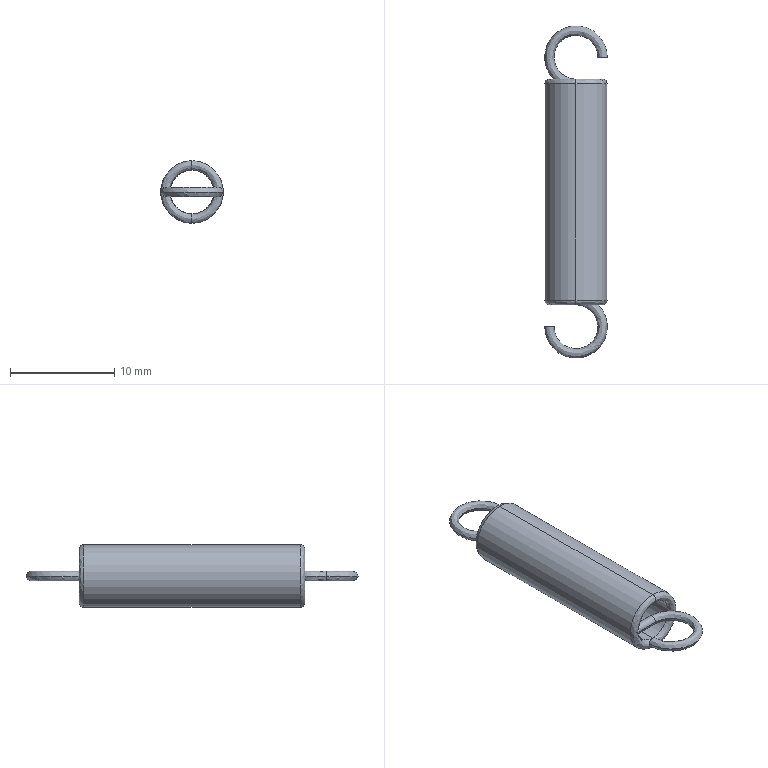Component | SolidWorks | YAWF-D6-L30-1 | 1 solid | 18 faces | box 6 x 31.8 x 6 mm | volume 327 mm3 | spline 8 | cylinder 8 | plane 2 | commonest cylinder face diameters 0.9 x4 6 x2 4.2 x2 | material Purchased Part
STEP:
#1=CARTESIAN_POINT('',(-2.205,-1.423,-0.001969));
#2=VERTEX_POINT('',#1);
#3=CARTESIAN_POINT('',(-2.124,-1.423,0.06299));
#4=VERTEX_POINT('',#3);
#5=CARTESIAN_POINT('',(-2.124,-1.423,-0.01969));
#6=DIRECTION('',(-0.,1.,-0.));
#7=DIRECTION('',(0.,0.,-1.));
#8=AXIS2_PLACEMENT_3D('',#5,#6,#7);
#9=CIRCLE('',#8,0.08268);
#10=EDGE_CURVE('',#2,#4,#9,.T.);
#11=ORIENTED_EDGE('',*,*,#10,.T.);
#12=CARTESIAN_POINT('',(-2.124,-1.423,0.09843));
#13=VERTEX_POINT('',#12);
#14=CARTESIAN_POINT('',(-2.124,-1.423,0.08071));
#15=DIRECTION('',(-1.,-0.,0.));
#16=DIRECTION('',(0.,0.,1.));
#17=AXIS2_PLACEMENT_3D('',#14,#15,#16);
#18=CIRCLE('',#17,0.01772);
#19=EDGE_CURVE('',#4,#13,#18,.T.);
#20=ORIENTED_EDGE('',*,*,#19,.T.);
#21=CARTESIAN_POINT('',(-2.124,-1.423,-0.1378));
#22=VERTEX_POINT('',#21);
#23=CARTESIAN_POINT('',(-2.124,-1.423,-0.01969));
#24=DIRECTION('',(-0.,1.,-0.));
#25=DIRECTION('',(0.,0.,1.));
#26=AXIS2_PLACEMENT_3D('',#23,#24,#25);
#27=CIRCLE('',#26,0.1181);
#28=EDGE_CURVE('',#22,#13,#27,.T.);
#29=ORIENTED_EDGE('',*,*,#28,.F.);
#30=CARTESIAN_POINT('',(-2.124,-1.423,-0.1024));
#31=VERTEX_POINT('',#30);
#32=CARTESIAN_POINT('',(-2.124,-1.423,-0.1201));
#33=DIRECTION('',(1.,-0.,0.));
#34=DIRECTION('',(0.,0.,-1.));
#35=AXIS2_PLACEMENT_3D('',#32,#33,#34);
#36=CIRCLE('',#35,0.01772);
#37=EDGE_CURVE('',#31,#22,#36,.T.);
#38=ORIENTED_EDGE('',*,*,#37,.F.);
#39=CARTESIAN_POINT('',(-2.205,-1.423,-0.0374));
#40=VERTEX_POINT('',#39);
#41=CARTESIAN_POINT('',(-2.124,-1.423,-0.01969));
#42=DIRECTION('',(-0.,1.,-0.));
#43=DIRECTION('',(0.,0.,-1.));
#44=AXIS2_PLACEMENT_3D('',#41,#42,#43);
#45=CIRCLE('',#44,0.08268);
#46=EDGE_CURVE('',#31,#40,#45,.T.);
#47=ORIENTED_EDGE('',*,*,#46,.T.);
#48=CARTESIAN_POINT('',(-2.224,-1.441,-0.01969));
#49=VERTEX_POINT('',#48);
#50=CARTESIAN_POINT('',(-2.205,-1.423,-0.0374));
#51=CARTESIAN_POINT('',(-2.205,-1.425,-0.0374));
#52=CARTESIAN_POINT('',(-2.205,-1.426,-0.03725));
#53=CARTESIAN_POINT('',(-2.206,-1.428,-0.03677));
#54=CARTESIAN_POINT('',(-2.206,-1.429,-0.03657));
#55=CARTESIAN_POINT('',(-2.206,-1.43,-0.03621));
#56=CARTESIAN_POINT('',(-2.206,-1.43,-0.03602));
#57=CARTESIAN_POINT('',(-2.207,-1.431,-0.03579));
#58=CARTESIAN_POINT('',(-2.207,-1.431,-0.03564));
#59=CARTESIAN_POINT('',(-2.207,-1.431,-0.03554));
#60=CARTESIAN_POINT('',(-2.208,-1.432,-0.03501));
#61=CARTESIAN_POINT('',(-2.208,-1.433,-0.03443));
#62=CARTESIAN_POINT('',(-2.21,-1.435,-0.03335));
#63=CARTESIAN_POINT('',(-2.21,-1.435,-0.03296));
#64=CARTESIAN_POINT('',(-2.211,-1.436,-0.03231));
#65=CARTESIAN_POINT('',(-2.211,-1.436,-0.03198));
#66=CARTESIAN_POINT('',(-2.212,-1.436,-0.03156));
#67=CARTESIAN_POINT('',(-2.212,-1.437,-0.03137));
#68=CARTESIAN_POINT('',(-2.212,-1.437,-0.03125));
#69=CARTESIAN_POINT('',(-2.212,-1.437,-0.03116));
#70=CARTESIAN_POINT('',(-2.213,-1.437,-0.03059));
#71=CARTESIAN_POINT('',(-2.214,-1.438,-0.02989));
#72=CARTESIAN_POINT('',(-2.215,-1.439,-0.02855));
#73=CARTESIAN_POINT('',(-2.216,-1.439,-0.02805));
#74=CARTESIAN_POINT('',(-2.217,-1.439,-0.02695));
#75=CARTESIAN_POINT('',(-2.218,-1.44,-0.0263));
#76=CARTESIAN_POINT('',(-2.221,-1.441,-0.02323));
#77=CARTESIAN_POINT('',(-2.223,-1.441,-0.02116));
#78=CARTESIAN_POINT('',(-2.224,-1.441,-0.01969));
#79=B_SPLINE_CURVE_WITH_KNOTS('',3,(#50,#51,#52,#53,#54,#55,#56,#57,#58,#59,#60,#61,#62,#63,#64,#65,#66,#67,#68,#69,#70,#71,#72,#73,#74,#75,#76,#77,#78),.UNSPECIFIED.,.F.,.F.,(4,2,2,1,2,2,2,2,1,1,2,2,2,2,2,4),(0.,0.125,0.1875,0.2187,0.2344,0.25,0.375,0.4375,0.4687,0.4844,0.4922,0.5,0.625,0.6875,0.75,1.),.UNSPECIFIED.);
#80=EDGE_CURVE('',#40,#49,#79,.T.);
#81=ORIENTED_EDGE('',*,*,#80,.T.);
#82=CARTESIAN_POINT('',(-2.224,-1.441,-0.01969));
#83=CARTESIAN_POINT('',(-2.224,-1.441,-0.01895));
#84=CARTESIAN_POINT('',(-2.223,-1.441,-0.01806));
#85=CARTESIAN_POINT('',(-2.221,-1.441,-0.01655));
#86=CARTESIAN_POINT('',(-2.221,-1.441,-0.01602));
#87=CARTESIAN_POINT('',(-2.219,-1.44,-0.01489));
#88=CARTESIAN_POINT('',(-2.219,-1.44,-0.01436));
#89=CARTESIAN_POINT('',(-2.217,-1.439,-0.01236));
#90=CARTESIAN_POINT('',(-2.216,-1.439,-0.01127));
#91=CARTESIAN_POINT('',(-2.214,-1.438,-0.009926));
#92=CARTESIAN_POINT('',(-2.214,-1.438,-0.009528));
#93=CARTESIAN_POINT('',(-2.213,-1.437,-0.009001));
#94=CARTESIAN_POINT('',(-2.213,-1.437,-0.008755));
#95=CARTESIAN_POINT('',(-2.213,-1.437,-0.008497));
#96=CARTESIAN_POINT('',(-2.212,-1.437,-0.008393));
#97=CARTESIAN_POINT('',(-2.212,-1.437,-0.008325));
#98=CARTESIAN_POINT('',(-2.212,-1.437,-0.008322));
#99=CARTESIAN_POINT('',(-2.211,-1.436,-0.007245));
#100=CARTESIAN_POINT('',(-2.21,-1.435,-0.006391));
#101=CARTESIAN_POINT('',(-2.209,-1.434,-0.005311));
#102=CARTESIAN_POINT('',(-2.208,-1.433,-0.004985));
#103=CARTESIAN_POINT('',(-2.208,-1.432,-0.004543));
#104=CARTESIAN_POINT('',(-2.208,-1.432,-0.004334));
#105=CARTESIAN_POINT('',(-2.207,-1.432,-0.004142));
#106=CARTESIAN_POINT('',(-2.207,-1.432,-0.004018));
#107=CARTESIAN_POINT('',(-2.207,-1.431,-0.003982));
#108=CARTESIAN_POINT('',(-2.206,-1.429,-0.002578));
#109=CARTESIAN_POINT('',(-2.205,-1.426,-0.001969));
#110=CARTESIAN_POINT('',(-2.205,-1.423,-0.001969));
#111=B_SPLINE_CURVE_WITH_KNOTS('',3,(#82,#83,#84,#85,#86,#87,#88,#89,#90,#91,#92,#93,#94,#95,#96,#97,#98,#99,#100,#101,#102,#103,#104,#105,#106,#107,#108,#109,#110),.UNSPECIFIED.,.F.,.F.,(4,2,2,2,2,2,1,1,2,2,2,2,1,2,2,4),(0.,0.125,0.1875,0.25,0.375,0.4375,0.4688,0.4844,0.4922,0.5,0.625,0.6875,0.7188,0.7344,0.75,1.),.UNSPECIFIED.);
#112=EDGE_CURVE('',#49,#2,#111,.T.);
#113=ORIENTED_EDGE('',*,*,#112,.T.);
#114=EDGE_LOOP('',(#11,#20,#29,#38,#47,#81,#113));
#115=FACE_OUTER_BOUND('',#114,.T.);
#116=CARTESIAN_POINT('',(-2.124,-1.423,0.06299));
#117=CARTESIAN_POINT('',(-2.289,-1.423,0.06299));
#118=CARTESIAN_POINT('',(-2.289,-1.423,-0.1024));
#119=CARTESIAN_POINT('',(-2.124,-1.423,-0.1024));
#120=CARTESIAN_POINT('',(-2.124,-1.434,0.06299));
#121=CARTESIAN_POINT('',(-2.289,-1.434,0.06299));
#122=CARTESIAN_POINT('',(-2.289,-1.434,-0.1024));
#123=CARTESIAN_POINT('',(-2.124,-1.434,-0.1024));
#124=CARTESIAN_POINT('',(-2.124,-1.441,0.07033));
#125=CARTESIAN_POINT('',(-2.304,-1.441,0.07033));
#126=CARTESIAN_POINT('',(-2.304,-1.441,-0.1097));
#127=CARTESIAN_POINT('',(-2.124,-1.441,-0.1097));
#128=CARTESIAN_POINT('',(-2.124,-1.441,0.08071));
#129=CARTESIAN_POINT('',(-2.325,-1.441,0.08071));
#130=CARTESIAN_POINT('',(-2.325,-1.441,-0.1201));
#131=CARTESIAN_POINT('',(-2.124,-1.441,-0.1201));
#132=CARTESIAN_POINT('',(-2.124,-1.441,0.09109));
#133=CARTESIAN_POINT('',(-2.346,-1.441,0.09109));
#134=CARTESIAN_POINT('',(-2.346,-1.441,-0.1305));
#135=CARTESIAN_POINT('',(-2.124,-1.441,-0.1305));
#136=CARTESIAN_POINT('',(-2.124,-1.434,0.09843));
#137=CARTESIAN_POINT('',(-2.36,-1.434,0.09843));
#138=CARTESIAN_POINT('',(-2.36,-1.434,-0.1378));
#139=CARTESIAN_POINT('',(-2.124,-1.434,-0.1378));
#140=CARTESIAN_POINT('',(-2.124,-1.423,0.09843));
#141=CARTESIAN_POINT('',(-2.36,-1.423,0.09843));
#142=CARTESIAN_POINT('',(-2.36,-1.423,-0.1378));
#143=CARTESIAN_POINT('',(-2.124,-1.423,-0.1378));
#144=(BOUNDED_SURFACE()B_SPLINE_SURFACE(3,3,((#116,#117,#118,#119),(#120,#121,#122,#123),(#124,#125,#126,#127),(#128,#129,#130,#131),(#132,#133,#134,#135),(#136,#137,#138,#139),(#140,#141,#142,#143)),.UNSPECIFIED.,.F.,.F.,.F.)B_SPLINE_SURFACE_WITH_KNOTS((4,3,4),(4,4),(0.,0.5,1.),(0.,1.),.UNSPECIFIED.)GEOMETRIC_REPRESENTATION_ITEM()RATIONAL_B_SPLINE_SURFACE(((1.,0.3333,0.3333,1.),(0.8047,0.2682,0.2682,0.8047),(0.8047,0.2682,0.2682,0.8047),(1.,0.3333,0.3333,1.),(0.8047,0.2682,0.2682,0.8047),(0.8047,0.2682,0.2682,0.8047),(1.,0.3333,0.3333,1.)))REPRESENTATION_ITEM('')SURFACE());
#145=ADVANCED_FACE('',(#115),#144,.T.);
#146=CARTESIAN_POINT('',(-2.124,-0.6083,0.09843));
#147=VERTEX_POINT('',#146);
#148=CARTESIAN_POINT('',(-2.124,-0.6083,-0.1378));
#149=VERTEX_POINT('',#148);
#150=CARTESIAN_POINT('',(-2.124,-0.6083,-0.01969));
#151=DIRECTION('',(0.,-1.,0.));
#152=DIRECTION('',(0.,0.,1.));
#153=AXIS2_PLACEMENT_3D('',#150,#151,#152);
#154=CIRCLE('',#153,0.1181);
#155=EDGE_CURVE('',#147,#149,#154,.T.);
#156=ORIENTED_EDGE('',*,*,#155,.F.);
#157=CARTESIAN_POINT('',(-2.124,-0.6083,0.06299));
#158=VERTEX_POINT('',#157);
#159=CARTESIAN_POINT('',(-2.124,-0.6083,0.08071));
#160=DIRECTION('',(-1.,-0.,0.));
#161=DIRECTION('',(0.,0.,1.));
#162=AXIS2_PLACEMENT_3D('',#159,#160,#161);
#163=CIRCLE('',#162,0.01772);
#164=EDGE_CURVE('',#147,#158,#163,.T.);
#165=ORIENTED_EDGE('',*,*,#164,.T.);
#166=CARTESIAN_POINT('',(-2.124,-0.6083,-0.1024));
#167=VERTEX_POINT('',#166);
#168=CARTESIAN_POINT('',(-2.124,-0.6083,-0.01969));
#169=DIRECTION('',(0.,-1.,0.));
#170=DIRECTION('',(0.,0.,-1.));
#171=AXIS2_PLACEMENT_3D('',#168,#169,#170);
#172=CIRCLE('',#171,0.08268);
#173=EDGE_CURVE('',#158,#167,#172,.T.);
#174=ORIENTED_EDGE('',*,*,#173,.T.);
#175=CARTESIAN_POINT('',(-2.124,-0.6083,-0.1201));
#176=DIRECTION('',(1.,-0.,0.));
#177=DIRECTION('',(0.,0.,-1.));
#178=AXIS2_PLACEMENT_3D('',#175,#176,#177);
#179=CIRCLE('',#178,0.01772);
#180=EDGE_CURVE('',#149,#167,#179,.T.);
#181=ORIENTED_EDGE('',*,*,#180,.F.);
#182=EDGE_LOOP('',(#156,#165,#174,#181));
#183=FACE_OUTER_BOUND('',#182,.T.);
#184=CARTESIAN_POINT('',(-2.124,-0.6083,0.09843));
#185=CARTESIAN_POINT('',(-2.36,-0.6083,0.09843));
#186=CARTESIAN_POINT('',(-2.36,-0.6083,-0.1378));
#187=CARTESIAN_POINT('',(-2.124,-0.6083,-0.1378));
#188=CARTESIAN_POINT('',(-2.124,-0.5728,0.09843));
#189=CARTESIAN_POINT('',(-2.36,-0.5728,0.09843));
#190=CARTESIAN_POINT('',(-2.36,-0.5728,-0.1378));
#191=CARTESIAN_POINT('',(-2.124,-0.5728,-0.1378));
#192=CARTESIAN_POINT('',(-2.124,-0.5728,0.06299));
#193=CARTESIAN_POINT('',(-2.289,-0.5728,0.06299));
#194=CARTESIAN_POINT('',(-2.289,-0.5728,-0.1024));
#195=CARTESIAN_POINT('',(-2.124,-0.5728,-0.1024));
#196=CARTESIAN_POINT('',(-2.124,-0.6083,0.06299));
#197=CARTESIAN_POINT('',(-2.289,-0.6083,0.06299));
#198=CARTESIAN_POINT('',(-2.289,-0.6083,-0.1024));
#199=CARTESIAN_POINT('',(-2.124,-0.6083,-0.1024));
#200=(BOUNDED_SURFACE()B_SPLINE_SURFACE(3,3,((#184,#185,#186,#187),(#188,#189,#190,#191),(#192,#193,#194,#195),(#196,#197,#198,#199)),.UNSPECIFIED.,.F.,.F.,.T.)B_SPLINE_SURFACE_WITH_KNOTS((4,4),(4,4),(0.,1.),(0.,1.),.UNSPECIFIED.)GEOMETRIC_REPRESENTATION_ITEM()RATIONAL_B_SPLINE_SURFACE(((1.,0.3333,0.3333,1.),(0.3333,0.1111,0.1111,0.3333),(0.3333,0.1111,0.1111,0.3333),(1.,0.3333,0.3333,1.)))REPRESENTATION_ITEM('')SURFACE());
#201=ADVANCED_FACE('',(#183),#200,.T.);
#202=CARTESIAN_POINT('',(-2.124,-1.423,-0.01969));
#203=DIRECTION('',(-0.,1.,-0.));
#204=DIRECTION('',(0.,0.,1.));
#205=AXIS2_PLACEMENT_3D('',#202,#203,#204);
#206=CIRCLE('',#205,0.1181);
#207=EDGE_CURVE('',#13,#22,#206,.T.);
#208=ORIENTED_EDGE('',*,*,#207,.T.);
#209=CARTESIAN_POINT('',(-2.124,-1.441,-0.1378));
#210=DIRECTION('',(-0.,1.,-0.));
#211=VECTOR('',#210,39.37);
#212=LINE('',#209,#211);
#213=EDGE_CURVE('',#22,#149,#212,.T.);
#214=ORIENTED_EDGE('',*,*,#213,.T.);
#215=CARTESIAN_POINT('',(-2.124,-0.6083,-0.01969));
#216=DIRECTION('',(0.,-1.,0.));
#217=DIRECTION('',(0.,0.,1.));
#218=AXIS2_PLACEMENT_3D('',#215,#216,#217);
#219=CIRCLE('',#218,0.1181);
#220=EDGE_CURVE('',#149,#147,#219,.T.);
#221=ORIENTED_EDGE('',*,*,#220,.T.);
#222=CARTESIAN_POINT('',(-2.124,-1.441,0.09843));
#223=DIRECTION('',(-0.,1.,-0.));
#224=VECTOR('',#223,39.37);
#225=LINE('',#222,#224);
#226=EDGE_CURVE('',#13,#147,#225,.T.);
#227=ORIENTED_EDGE('',*,*,#226,.F.);
#228=EDGE_LOOP('',(#208,#214,#221,#227));
#229=FACE_OUTER_BOUND('',#228,.T.);
#230=CARTESIAN_POINT('',(-2.124,-1.441,-0.01969));
#231=DIRECTION('',(-0.,1.,-0.));
#232=DIRECTION('',(0.,0.,1.));
#233=AXIS2_PLACEMENT_3D('',#230,#231,#232);
#234=CYLINDRICAL_SURFACE('',#233,0.1181);
#235=ADVANCED_FACE('',(#229),#234,.T.);
#236=ORIENTED_EDGE('',*,*,#112,.F.);
#237=CARTESIAN_POINT('',(-2.124,-1.441,-0.01969));
#238=VERTEX_POINT('',#237);
#239=CARTESIAN_POINT('',(-2.224,-1.441,-0.01969));
#240=DIRECTION('',(1.,-0.,0.));
#241=VECTOR('',#240,39.37);
#242=LINE('',#239,#241);
#243=EDGE_CURVE('',#49,#238,#242,.T.);
#244=ORIENTED_EDGE('',*,*,#243,.T.);
#245=CARTESIAN_POINT('',(-2.124,-1.406,-0.01969));
#246=VERTEX_POINT('',#245);
#247=CARTESIAN_POINT('',(-2.124,-1.423,-0.01969));
#248=DIRECTION('',(-1.,0.,-0.));
#249=DIRECTION('',(0.,1.,0.));
#250=AXIS2_PLACEMENT_3D('',#247,#248,#249);
#251=CIRCLE('',#250,0.01772);
#252=EDGE_CURVE('',#238,#246,#251,.T.);
#253=ORIENTED_EDGE('',*,*,#252,.T.);
#254=CARTESIAN_POINT('',(-2.207,-1.406,-0.01969));
#255=VERTEX_POINT('',#254);
#256=CARTESIAN_POINT('',(-2.224,-1.406,-0.01969));
#257=DIRECTION('',(1.,-0.,0.));
#258=VECTOR('',#257,39.37);
#259=LINE('',#256,#258);
#260=EDGE_CURVE('',#255,#246,#259,.T.);
#261=ORIENTED_EDGE('',*,*,#260,.F.);
#262=CARTESIAN_POINT('',(-2.207,-1.406,-0.01969));
#263=CARTESIAN_POINT('',(-2.207,-1.406,-0.01505));
#264=CARTESIAN_POINT('',(-2.206,-1.407,-0.01045));
#265=CARTESIAN_POINT('',(-2.205,-1.414,-0.00387));
#266=CARTESIAN_POINT('',(-2.205,-1.419,-0.001969));
#267=CARTESIAN_POINT('',(-2.205,-1.423,-0.001969));
#268=B_SPLINE_CURVE_WITH_KNOTS('',3,(#262,#263,#264,#265,#266,#267),.UNSPECIFIED.,.F.,.F.,(4,2,4),(0.0007057,0.001058,0.001411),.UNSPECIFIED.);
#269=EDGE_CURVE('',#255,#2,#268,.T.);
#270=ORIENTED_EDGE('',*,*,#269,.T.);
#271=EDGE_LOOP('',(#236,#244,#253,#261,#270));
#272=FACE_OUTER_BOUND('',#271,.T.);
#273=CARTESIAN_POINT('',(-2.224,-1.423,-0.01969));
#274=DIRECTION('',(1.,-0.,0.));
#275=DIRECTION('',(0.,1.,0.));
#276=AXIS2_PLACEMENT_3D('',#273,#274,#275);
#277=CYLINDRICAL_SURFACE('',#276,0.01772);
#278=ADVANCED_FACE('',(#272),#277,.T.);
#279=ORIENTED_EDGE('',*,*,#46,.F.);
#280=CARTESIAN_POINT('',(-2.124,-1.441,-0.1024));
#281=DIRECTION('',(-0.,1.,-0.));
#282=VECTOR('',#281,39.37);
#283=LINE('',#280,#282);
#284=EDGE_CURVE('',#31,#167,#283,.T.);
#285=ORIENTED_EDGE('',*,*,#284,.T.);
#286=ORIENTED_EDGE('',*,*,#173,.F.);
#287=CARTESIAN_POINT('',(-2.124,-1.441,0.06299));
#288=DIRECTION('',(-0.,1.,-0.));
#289=VECTOR('',#288,39.37);
#290=LINE('',#287,#289);
#291=EDGE_CURVE('',#4,#158,#290,.T.);
#292=ORIENTED_EDGE('',*,*,#291,.F.);
#293=ORIENTED_EDGE('',*,*,#10,.F.);
#294=ORIENTED_EDGE('',*,*,#269,.F.);
#295=CARTESIAN_POINT('',(-2.205,-1.423,-0.0374));
#296=CARTESIAN_POINT('',(-2.205,-1.419,-0.0374));
#297=CARTESIAN_POINT('',(-2.205,-1.414,-0.03547));
#298=CARTESIAN_POINT('',(-2.206,-1.407,-0.02895));
#299=CARTESIAN_POINT('',(-2.207,-1.406,-0.02432));
#300=CARTESIAN_POINT('',(-2.207,-1.406,-0.01969));
#301=B_SPLINE_CURVE_WITH_KNOTS('',3,(#295,#296,#297,#298,#299,#300),.UNSPECIFIED.,.F.,.F.,(4,2,4),(0.,0.0003528,0.0007057),.UNSPECIFIED.);
#302=EDGE_CURVE('',#40,#255,#301,.T.);
#303=ORIENTED_EDGE('',*,*,#302,.F.);
#304=EDGE_LOOP('',(#279,#285,#286,#292,#293,#294,#303));
#305=FACE_OUTER_BOUND('',#304,.T.);
#306=CARTESIAN_POINT('',(-2.124,-1.441,-0.01969));
#307=DIRECTION('',(-0.,1.,-0.));
#308=DIRECTION('',(0.,0.,1.));
#309=AXIS2_PLACEMENT_3D('',#306,#307,#308);
#310=CYLINDRICAL_SURFACE('',#309,0.08268);
#311=ADVANCED_FACE('',(#305),#310,.F.);
#312=CARTESIAN_POINT('',(-2.124,-0.5906,-0.01969));
#313=VERTEX_POINT('',#312);
#314=CARTESIAN_POINT('',(-2.124,-0.626,-0.01969));
#315=VERTEX_POINT('',#314);
#316=CARTESIAN_POINT('',(-2.124,-0.6083,-0.01969));
#317=DIRECTION('',(1.,-0.,0.));
#318=DIRECTION('',(0.,1.,0.));
#319=AXIS2_PLACEMENT_3D('',#316,#317,#318);
#320=CIRCLE('',#319,0.01772);
#321=EDGE_CURVE('',#313,#315,#320,.T.);
#322=ORIENTED_EDGE('',*,*,#321,.T.);
#323=CARTESIAN_POINT('',(-2.041,-0.626,-0.01969));
#324=VERTEX_POINT('',#323);
#325=CARTESIAN_POINT('',(-2.124,-0.626,-0.01969));
#326=DIRECTION('',(1.,-0.,0.));
#327=VECTOR('',#326,39.37);
#328=LINE('',#325,#327);
#329=EDGE_CURVE('',#315,#324,#328,.T.);
#330=ORIENTED_EDGE('',*,*,#329,.T.);
#331=CARTESIAN_POINT('',(-2.043,-0.6083,-0.001969));
#332=VERTEX_POINT('',#331);
#333=CARTESIAN_POINT('',(-2.041,-0.626,-0.01969));
#334=CARTESIAN_POINT('',(-2.041,-0.626,-0.01505));
#335=CARTESIAN_POINT('',(-2.042,-0.6241,-0.01045));
#336=CARTESIAN_POINT('',(-2.043,-0.6175,-0.00387));
#337=CARTESIAN_POINT('',(-2.043,-0.613,-0.001969));
#338=CARTESIAN_POINT('',(-2.043,-0.6083,-0.001969));
#339=B_SPLINE_CURVE_WITH_KNOTS('',3,(#333,#334,#335,#336,#337,#338),.UNSPECIFIED.,.F.,.F.,(4,2,4),(0.0007057,0.001058,0.001411),.UNSPECIFIED.);
#340=EDGE_CURVE('',#324,#332,#339,.T.);
#341=ORIENTED_EDGE('',*,*,#340,.T.);
#342=CARTESIAN_POINT('',(-2.024,-0.5906,-0.01969));
#343=VERTEX_POINT('',#342);
#344=CARTESIAN_POINT('',(-2.024,-0.5906,-0.01969));
#345=CARTESIAN_POINT('',(-2.024,-0.5906,-0.01895));
#346=CARTESIAN_POINT('',(-2.025,-0.5906,-0.01806));
#347=CARTESIAN_POINT('',(-2.027,-0.5908,-0.01655));
#348=CARTESIAN_POINT('',(-2.027,-0.5909,-0.01602));
#349=CARTESIAN_POINT('',(-2.029,-0.5912,-0.01489));
#350=CARTESIAN_POINT('',(-2.029,-0.5914,-0.01436));
#351=CARTESIAN_POINT('',(-2.031,-0.5921,-0.01236));
#352=CARTESIAN_POINT('',(-2.032,-0.5926,-0.01127));
#353=CARTESIAN_POINT('',(-2.034,-0.5935,-0.009926));
#354=CARTESIAN_POINT('',(-2.034,-0.5937,-0.009528));
#355=CARTESIAN_POINT('',(-2.035,-0.5941,-0.009001));
#356=CARTESIAN_POINT('',(-2.035,-0.5943,-0.008755));
#357=CARTESIAN_POINT('',(-2.036,-0.5945,-0.008497));
#358=CARTESIAN_POINT('',(-2.036,-0.5946,-0.008393));
#359=CARTESIAN_POINT('',(-2.036,-0.5947,-0.008325));
#360=CARTESIAN_POINT('',(-2.036,-0.5947,-0.008322));
#361=CARTESIAN_POINT('',(-2.037,-0.5956,-0.007245));
#362=CARTESIAN_POINT('',(-2.038,-0.5965,-0.006391));
#363=CARTESIAN_POINT('',(-2.039,-0.5979,-0.005311));
#364=CARTESIAN_POINT('',(-2.04,-0.5984,-0.004985));
#365=CARTESIAN_POINT('',(-2.04,-0.5991,-0.004543));
#366=CARTESIAN_POINT('',(-2.04,-0.5994,-0.004334));
#367=CARTESIAN_POINT('',(-2.041,-0.5998,-0.004142));
#368=CARTESIAN_POINT('',(-2.041,-0.6,-0.004018));
#369=CARTESIAN_POINT('',(-2.041,-0.6001,-0.003982));
#370=CARTESIAN_POINT('',(-2.042,-0.6028,-0.002578));
#371=CARTESIAN_POINT('',(-2.043,-0.6056,-0.001969));
#372=CARTESIAN_POINT('',(-2.043,-0.6083,-0.001969));
#373=B_SPLINE_CURVE_WITH_KNOTS('',3,(#344,#345,#346,#347,#348,#349,#350,#351,#352,#353,#354,#355,#356,#357,#358,#359,#360,#361,#362,#363,#364,#365,#366,#367,#368,#369,#370,#371,#372),.UNSPECIFIED.,.F.,.F.,(4,2,2,2,2,2,1,1,2,2,2,2,1,2,2,4),(0.,0.125,0.1875,0.25,0.375,0.4375,0.4688,0.4844,0.4922,0.5,0.625,0.6875,0.7188,0.7344,0.75,1.),.UNSPECIFIED.);
#374=EDGE_CURVE('',#343,#332,#373,.T.);
#375=ORIENTED_EDGE('',*,*,#374,.F.);
#376=CARTESIAN_POINT('',(-2.124,-0.5906,-0.01969));
#377=DIRECTION('',(1.,-0.,0.));
#378=VECTOR('',#377,39.37);
#379=LINE('',#376,#378);
#380=EDGE_CURVE('',#313,#343,#379,.T.);
#381=ORIENTED_EDGE('',*,*,#380,.F.);
#382=EDGE_LOOP('',(#322,#330,#341,#375,#381));
#383=FACE_OUTER_BOUND('',#382,.T.);
#384=CARTESIAN_POINT('',(-2.124,-0.6083,-0.01969));
#385=DIRECTION('',(1.,-0.,0.));
#386=DIRECTION('',(0.,1.,0.));
#387=AXIS2_PLACEMENT_3D('',#384,#385,#386);
#388=CYLINDRICAL_SURFACE('',#387,0.01772);
#389=ADVANCED_FACE('',(#383),#388,.T.);
#390=ORIENTED_EDGE('',*,*,#252,.F.);
#391=CARTESIAN_POINT('',(-2.207,-1.524,-0.01969));
#392=VERTEX_POINT('',#391);
#393=CARTESIAN_POINT('',(-2.124,-1.524,-0.01969));
#394=DIRECTION('',(-0.,0.,-1.));
#395=DIRECTION('',(0.,1.,0.));
#396=AXIS2_PLACEMENT_3D('',#393,#394,#395);
#397=CIRCLE('',#396,0.08268);
#398=EDGE_CURVE('',#238,#392,#397,.T.);
#399=ORIENTED_EDGE('',*,*,#398,.T.);
#400=CARTESIAN_POINT('',(-2.242,-1.524,-0.01969));
#401=VERTEX_POINT('',#400);
#402=CARTESIAN_POINT('',(-2.207,-1.524,-0.01969));
#403=CARTESIAN_POINT('',(-2.207,-1.524,-0.01501));
#404=CARTESIAN_POINT('',(-2.209,-1.524,-0.01043));
#405=CARTESIAN_POINT('',(-2.215,-1.524,-0.003886));
#406=CARTESIAN_POINT('',(-2.22,-1.524,-0.001965));
#407=CARTESIAN_POINT('',(-2.229,-1.524,-0.001972));
#408=CARTESIAN_POINT('',(-2.234,-1.524,-0.003896));
#409=CARTESIAN_POINT('',(-2.24,-1.524,-0.01044));
#410=CARTESIAN_POINT('',(-2.242,-1.524,-0.01506));
#411=CARTESIAN_POINT('',(-2.242,-1.524,-0.01969));
#412=B_SPLINE_CURVE_WITH_KNOTS('',3,(#402,#403,#404,#405,#406,#407,#408,#409,#410,#411),.UNSPECIFIED.,.F.,.F.,(4,2,2,2,4),(0.002111,0.002462,0.002814,0.003165,0.003517),.UNSPECIFIED.);
#413=EDGE_CURVE('',#392,#401,#412,.T.);
#414=ORIENTED_EDGE('',*,*,#413,.T.);
#415=CARTESIAN_POINT('',(-2.124,-1.524,-0.01969));
#416=DIRECTION('',(-0.,0.,-1.));
#417=DIRECTION('',(0.,1.,0.));
#418=AXIS2_PLACEMENT_3D('',#415,#416,#417);
#419=CIRCLE('',#418,0.1181);
#420=EDGE_CURVE('',#246,#401,#419,.T.);
#421=ORIENTED_EDGE('',*,*,#420,.F.);
#422=EDGE_LOOP('',(#390,#399,#414,#421));
#423=FACE_OUTER_BOUND('',#422,.T.);
#424=CARTESIAN_POINT('',(-2.124,-1.406,-0.01969));
#425=CARTESIAN_POINT('',(-2.,-1.406,-0.01969));
#426=CARTESIAN_POINT('',(-1.953,-1.52,-0.01969));
#427=CARTESIAN_POINT('',(-2.04,-1.607,-0.01969));
#428=CARTESIAN_POINT('',(-2.128,-1.695,-0.01969));
#429=CARTESIAN_POINT('',(-2.242,-1.647,-0.01969));
#430=CARTESIAN_POINT('',(-2.242,-1.524,-0.01969));
#431=CARTESIAN_POINT('',(-2.124,-1.406,0.01575));
#432=CARTESIAN_POINT('',(-2.,-1.406,0.01575));
#433=CARTESIAN_POINT('',(-1.953,-1.52,0.01575));
#434=CARTESIAN_POINT('',(-2.04,-1.607,0.01575));
#435=CARTESIAN_POINT('',(-2.128,-1.695,0.01575));
#436=CARTESIAN_POINT('',(-2.242,-1.647,0.01575));
#437=CARTESIAN_POINT('',(-2.242,-1.524,0.01575));
#438=CARTESIAN_POINT('',(-2.124,-1.441,0.01575));
#439=CARTESIAN_POINT('',(-2.037,-1.441,0.01575));
#440=CARTESIAN_POINT('',(-2.004,-1.521,0.01575));
#441=CARTESIAN_POINT('',(-2.066,-1.582,0.01575));
#442=CARTESIAN_POINT('',(-2.127,-1.643,0.01575));
#443=CARTESIAN_POINT('',(-2.207,-1.61,0.01575));
#444=CARTESIAN_POINT('',(-2.207,-1.524,0.01575));
#445=CARTESIAN_POINT('',(-2.124,-1.441,-0.01969));
#446=CARTESIAN_POINT('',(-2.037,-1.441,-0.01969));
#447=CARTESIAN_POINT('',(-2.004,-1.521,-0.01969));
#448=CARTESIAN_POINT('',(-2.066,-1.582,-0.01969));
#449=CARTESIAN_POINT('',(-2.127,-1.643,-0.01969));
#450=CARTESIAN_POINT('',(-2.207,-1.61,-0.01969));
#451=CARTESIAN_POINT('',(-2.207,-1.524,-0.01969));
#452=(BOUNDED_SURFACE()B_SPLINE_SURFACE(3,3,((#424,#425,#426,#427,#428,#429,#430),(#431,#432,#433,#434,#435,#436,#437),(#438,#439,#440,#441,#442,#443,#444),(#445,#446,#447,#448,#449,#450,#451)),.UNSPECIFIED.,.F.,.F.,.F.)B_SPLINE_SURFACE_WITH_KNOTS((4,4),(4,3,4),(0.,1.),(0.,0.5,1.),.UNSPECIFIED.)GEOMETRIC_REPRESENTATION_ITEM()RATIONAL_B_SPLINE_SURFACE(((1.,0.5885,0.5885,1.,0.5885,0.5885,1.),(0.3333,0.1962,0.1962,0.3333,0.1962,0.1962,0.3333),(0.3333,0.1962,0.1962,0.3333,0.1962,0.1962,0.3333),(1.,0.5885,0.5885,1.,0.5885,0.5885,1.)))REPRESENTATION_ITEM('')SURFACE());
#453=ADVANCED_FACE('',(#423),#452,.T.);
#454=CARTESIAN_POINT('',(-2.006,-0.5079,-0.01969));
#455=VERTEX_POINT('',#454);
#456=CARTESIAN_POINT('',(-2.041,-0.5079,-0.01969));
#457=VERTEX_POINT('',#456);
#458=CARTESIAN_POINT('',(-2.006,-0.5079,-0.01969));
#459=CARTESIAN_POINT('',(-2.006,-0.5079,-0.02431));
#460=CARTESIAN_POINT('',(-2.008,-0.5079,-0.02891));
#461=CARTESIAN_POINT('',(-2.014,-0.5079,-0.03552));
#462=CARTESIAN_POINT('',(-2.019,-0.5079,-0.0374));
#463=CARTESIAN_POINT('',(-2.028,-0.5079,-0.0374));
#464=CARTESIAN_POINT('',(-2.033,-0.5079,-0.03548));
#465=CARTESIAN_POINT('',(-2.039,-0.5079,-0.02895));
#466=CARTESIAN_POINT('',(-2.041,-0.5079,-0.02436));
#467=CARTESIAN_POINT('',(-2.041,-0.5079,-0.01969));
#468=B_SPLINE_CURVE_WITH_KNOTS('',3,(#458,#459,#460,#461,#462,#463,#464,#465,#466,#467),.UNSPECIFIED.,.F.,.F.,(4,2,2,2,4),(0.0007036,0.001055,0.001407,0.001759,0.002111),.UNSPECIFIED.);
#469=EDGE_CURVE('',#455,#457,#468,.T.);
#470=ORIENTED_EDGE('',*,*,#469,.T.);
#471=CARTESIAN_POINT('',(-2.124,-0.5079,-0.01969));
#472=DIRECTION('',(0.,-0.,1.));
#473=DIRECTION('',(0.,-1.,-0.));
#474=AXIS2_PLACEMENT_3D('',#471,#472,#473);
#475=CIRCLE('',#474,0.08268);
#476=EDGE_CURVE('',#457,#313,#475,.T.);
#477=ORIENTED_EDGE('',*,*,#476,.T.);
#478=CARTESIAN_POINT('',(-2.124,-0.6083,-0.01969));
#479=DIRECTION('',(1.,-0.,0.));
#480=DIRECTION('',(0.,1.,0.));
#481=AXIS2_PLACEMENT_3D('',#478,#479,#480);
#482=CIRCLE('',#481,0.01772);
#483=EDGE_CURVE('',#315,#313,#482,.T.);
#484=ORIENTED_EDGE('',*,*,#483,.F.);
#485=CARTESIAN_POINT('',(-2.124,-0.5079,-0.01969));
#486=DIRECTION('',(0.,-0.,1.));
#487=DIRECTION('',(0.,-1.,-0.));
#488=AXIS2_PLACEMENT_3D('',#485,#486,#487);
#489=CIRCLE('',#488,0.1181);
#490=EDGE_CURVE('',#455,#315,#489,.T.);
#491=ORIENTED_EDGE('',*,*,#490,.F.);
#492=EDGE_LOOP('',(#470,#477,#484,#491));
#493=FACE_OUTER_BOUND('',#492,.T.);
#494=CARTESIAN_POINT('',(-2.006,-0.5079,-0.01969));
#495=CARTESIAN_POINT('',(-2.006,-0.3843,-0.01969));
#496=CARTESIAN_POINT('',(-2.12,-0.3369,-0.01969));
#497=CARTESIAN_POINT('',(-2.208,-0.4244,-0.01969));
#498=CARTESIAN_POINT('',(-2.295,-0.5118,-0.01969));
#499=CARTESIAN_POINT('',(-2.248,-0.626,-0.01969));
#500=CARTESIAN_POINT('',(-2.124,-0.626,-0.01969));
#501=CARTESIAN_POINT('',(-2.006,-0.5079,-0.05512));
#502=CARTESIAN_POINT('',(-2.006,-0.3843,-0.05512));
#503=CARTESIAN_POINT('',(-2.12,-0.3369,-0.05512));
#504=CARTESIAN_POINT('',(-2.208,-0.4244,-0.05512));
#505=CARTESIAN_POINT('',(-2.295,-0.5118,-0.05512));
#506=CARTESIAN_POINT('',(-2.248,-0.626,-0.05512));
#507=CARTESIAN_POINT('',(-2.124,-0.626,-0.05512));
#508=CARTESIAN_POINT('',(-2.041,-0.5079,-0.05512));
#509=CARTESIAN_POINT('',(-2.041,-0.4213,-0.05512));
#510=CARTESIAN_POINT('',(-2.121,-0.3882,-0.05512));
#511=CARTESIAN_POINT('',(-2.182,-0.4494,-0.05512));
#512=CARTESIAN_POINT('',(-2.244,-0.5106,-0.05512));
#513=CARTESIAN_POINT('',(-2.211,-0.5906,-0.05512));
#514=CARTESIAN_POINT('',(-2.124,-0.5906,-0.05512));
#515=CARTESIAN_POINT('',(-2.041,-0.5079,-0.01969));
#516=CARTESIAN_POINT('',(-2.041,-0.4213,-0.01969));
#517=CARTESIAN_POINT('',(-2.121,-0.3882,-0.01969));
#518=CARTESIAN_POINT('',(-2.182,-0.4494,-0.01969));
#519=CARTESIAN_POINT('',(-2.244,-0.5106,-0.01969));
#520=CARTESIAN_POINT('',(-2.211,-0.5906,-0.01969));
#521=CARTESIAN_POINT('',(-2.124,-0.5906,-0.01969));
#522=(BOUNDED_SURFACE()B_SPLINE_SURFACE(3,3,((#494,#495,#496,#497,#498,#499,#500),(#501,#502,#503,#504,#505,#506,#507),(#508,#509,#510,#511,#512,#513,#514),(#515,#516,#517,#518,#519,#520,#521)),.UNSPECIFIED.,.F.,.F.,.T.)B_SPLINE_SURFACE_WITH_KNOTS((4,4),(4,3,4),(0.,1.),(0.,0.5,1.),.UNSPECIFIED.)GEOMETRIC_REPRESENTATION_ITEM()RATIONAL_B_SPLINE_SURFACE(((1.,0.5885,0.5885,1.,0.5885,0.5885,1.),(0.3333,0.1962,0.1962,0.3333,0.1962,0.1962,0.3333),(0.3333,0.1962,0.1962,0.3333,0.1962,0.1962,0.3333),(1.,0.5885,0.5885,1.,0.5885,0.5885,1.)))REPRESENTATION_ITEM('')SURFACE());
#523=ADVANCED_FACE('',(#493),#522,.T.);
#524=ORIENTED_EDGE('',*,*,#213,.F.);
#525=ORIENTED_EDGE('',*,*,#28,.T.);
#526=ORIENTED_EDGE('',*,*,#226,.T.);
#527=ORIENTED_EDGE('',*,*,#155,.T.);
#528=EDGE_LOOP('',(#524,#525,#526,#527));
#529=FACE_OUTER_BOUND('',#528,.T.);
#530=CARTESIAN_POINT('',(-2.124,-1.441,-0.01969));
#531=DIRECTION('',(-0.,1.,-0.));
#532=DIRECTION('',(0.,0.,1.));
#533=AXIS2_PLACEMENT_3D('',#530,#531,#532);
#534=CYLINDRICAL_SURFACE('',#533,0.1181);
#535=ADVANCED_FACE('',(#529),#534,.T.);
#536=ORIENTED_EDGE('',*,*,#19,.F.);
#537=CARTESIAN_POINT('',(-2.124,-1.423,-0.01969));
#538=DIRECTION('',(-0.,1.,-0.));
#539=DIRECTION('',(0.,0.,-1.));
#540=AXIS2_PLACEMENT_3D('',#537,#538,#539);
#541=CIRCLE('',#540,0.08268);
#542=EDGE_CURVE('',#4,#31,#541,.T.);
#543=ORIENTED_EDGE('',*,*,#542,.T.);
#544=ORIENTED_EDGE('',*,*,#37,.T.);
#545=ORIENTED_EDGE('',*,*,#207,.F.);
#546=EDGE_LOOP('',(#536,#543,#544,#545));
#547=FACE_OUTER_BOUND('',#546,.T.);
#548=CARTESIAN_POINT('',(-2.124,-1.423,-0.1024));
#549=CARTESIAN_POINT('',(-1.959,-1.423,-0.1024));
#550=CARTESIAN_POINT('',(-1.959,-1.423,0.06299));
#551=CARTESIAN_POINT('',(-2.124,-1.423,0.06299));
#552=CARTESIAN_POINT('',(-2.124,-1.434,-0.1024));
#553=CARTESIAN_POINT('',(-1.959,-1.434,-0.1024));
#554=CARTESIAN_POINT('',(-1.959,-1.434,0.06299));
#555=CARTESIAN_POINT('',(-2.124,-1.434,0.06299));
#556=CARTESIAN_POINT('',(-2.124,-1.441,-0.1097));
#557=CARTESIAN_POINT('',(-1.944,-1.441,-0.1097));
#558=CARTESIAN_POINT('',(-1.944,-1.441,0.07033));
#559=CARTESIAN_POINT('',(-2.124,-1.441,0.07033));
#560=CARTESIAN_POINT('',(-2.124,-1.441,-0.1201));
#561=CARTESIAN_POINT('',(-1.923,-1.441,-0.1201));
#562=CARTESIAN_POINT('',(-1.923,-1.441,0.08071));
#563=CARTESIAN_POINT('',(-2.124,-1.441,0.08071));
#564=CARTESIAN_POINT('',(-2.124,-1.441,-0.1305));
#565=CARTESIAN_POINT('',(-1.902,-1.441,-0.1305));
#566=CARTESIAN_POINT('',(-1.902,-1.441,0.09109));
#567=CARTESIAN_POINT('',(-2.124,-1.441,0.09109));
#568=CARTESIAN_POINT('',(-2.124,-1.434,-0.1378));
#569=CARTESIAN_POINT('',(-1.888,-1.434,-0.1378));
#570=CARTESIAN_POINT('',(-1.888,-1.434,0.09843));
#571=CARTESIAN_POINT('',(-2.124,-1.434,0.09843));
#572=CARTESIAN_POINT('',(-2.124,-1.423,-0.1378));
#573=CARTESIAN_POINT('',(-1.888,-1.423,-0.1378));
#574=CARTESIAN_POINT('',(-1.888,-1.423,0.09843));
#575=CARTESIAN_POINT('',(-2.124,-1.423,0.09843));
#576=(BOUNDED_SURFACE()B_SPLINE_SURFACE(3,3,((#548,#549,#550,#551),(#552,#553,#554,#555),(#556,#557,#558,#559),(#560,#561,#562,#563),(#564,#565,#566,#567),(#568,#569,#570,#571),(#572,#573,#574,#575)),.UNSPECIFIED.,.F.,.F.,.F.)B_SPLINE_SURFACE_WITH_KNOTS((4,3,4),(4,4),(0.,0.5,1.),(0.,1.),.UNSPECIFIED.)GEOMETRIC_REPRESENTATION_ITEM()RATIONAL_B_SPLINE_SURFACE(((1.,0.3333,0.3333,1.),(0.8047,0.2682,0.2682,0.8047),(0.8047,0.2682,0.2682,0.8047),(1.,0.3333,0.3333,1.),(0.8047,0.2682,0.2682,0.8047),(0.8047,0.2682,0.2682,0.8047),(1.,0.3333,0.3333,1.)))REPRESENTATION_ITEM('')SURFACE());
#577=ADVANCED_FACE('',(#547),#576,.T.);
#578=ORIENTED_EDGE('',*,*,#164,.F.);
#579=ORIENTED_EDGE('',*,*,#220,.F.);
#580=ORIENTED_EDGE('',*,*,#180,.T.);
#581=CARTESIAN_POINT('',(-2.043,-0.6083,-0.0374));
#582=VERTEX_POINT('',#581);
#583=CARTESIAN_POINT('',(-2.124,-0.6083,-0.01969));
#584=DIRECTION('',(0.,-1.,0.));
#585=DIRECTION('',(0.,0.,-1.));
#586=AXIS2_PLACEMENT_3D('',#583,#584,#585);
#587=CIRCLE('',#586,0.08268);
#588=EDGE_CURVE('',#167,#582,#587,.T.);
#589=ORIENTED_EDGE('',*,*,#588,.T.);
#590=CARTESIAN_POINT('',(-2.043,-0.6083,-0.0374));
#591=CARTESIAN_POINT('',(-2.043,-0.6069,-0.0374));
#592=CARTESIAN_POINT('',(-2.043,-0.6056,-0.03725));
#593=CARTESIAN_POINT('',(-2.042,-0.6036,-0.03677));
#594=CARTESIAN_POINT('',(-2.042,-0.6029,-0.03657));
#595=CARTESIAN_POINT('',(-2.042,-0.6019,-0.03621));
#596=CARTESIAN_POINT('',(-2.042,-0.6014,-0.03602));
#597=CARTESIAN_POINT('',(-2.041,-0.6009,-0.03579));
#598=CARTESIAN_POINT('',(-2.041,-0.6006,-0.03564));
#599=CARTESIAN_POINT('',(-2.041,-0.6004,-0.03554));
#600=CARTESIAN_POINT('',(-2.04,-0.5993,-0.03501));
#601=CARTESIAN_POINT('',(-2.04,-0.5984,-0.03443));
#602=CARTESIAN_POINT('',(-2.038,-0.597,-0.03335));
#603=CARTESIAN_POINT('',(-2.038,-0.5965,-0.03296));
#604=CARTESIAN_POINT('',(-2.037,-0.5958,-0.03231));
#605=CARTESIAN_POINT('',(-2.037,-0.5955,-0.03198));
#606=CARTESIAN_POINT('',(-2.036,-0.5951,-0.03156));
#607=CARTESIAN_POINT('',(-2.036,-0.595,-0.03137));
#608=CARTESIAN_POINT('',(-2.036,-0.5948,-0.03125));
#609=CARTESIAN_POINT('',(-2.036,-0.5948,-0.03116));
#610=CARTESIAN_POINT('',(-2.035,-0.5943,-0.03059));
#611=CARTESIAN_POINT('',(-2.034,-0.5938,-0.02989));
#612=CARTESIAN_POINT('',(-2.033,-0.5929,-0.02855));
#613=CARTESIAN_POINT('',(-2.032,-0.5926,-0.02805));
#614=CARTESIAN_POINT('',(-2.031,-0.5921,-0.02695));
#615=CARTESIAN_POINT('',(-2.03,-0.5918,-0.0263));
#616=CARTESIAN_POINT('',(-2.027,-0.5907,-0.02323));
#617=CARTESIAN_POINT('',(-2.025,-0.5906,-0.02116));
#618=CARTESIAN_POINT('',(-2.024,-0.5906,-0.01969));
#619=B_SPLINE_CURVE_WITH_KNOTS('',3,(#590,#591,#592,#593,#594,#595,#596,#597,#598,#599,#600,#601,#602,#603,#604,#605,#606,#607,#608,#609,#610,#611,#612,#613,#614,#615,#616,#617,#618),.UNSPECIFIED.,.F.,.F.,(4,2,2,1,2,2,2,2,1,1,2,2,2,2,2,4),(0.,0.125,0.1875,0.2187,0.2344,0.25,0.375,0.4375,0.4687,0.4844,0.4922,0.5,0.625,0.6875,0.75,1.),.UNSPECIFIED.);
#620=EDGE_CURVE('',#582,#343,#619,.T.);
#621=ORIENTED_EDGE('',*,*,#620,.T.);
#622=ORIENTED_EDGE('',*,*,#374,.T.);
#623=CARTESIAN_POINT('',(-2.124,-0.6083,-0.01969));
#624=DIRECTION('',(0.,-1.,0.));
#625=DIRECTION('',(0.,0.,-1.));
#626=AXIS2_PLACEMENT_3D('',#623,#624,#625);
#627=CIRCLE('',#626,0.08268);
#628=EDGE_CURVE('',#332,#158,#627,.T.);
#629=ORIENTED_EDGE('',*,*,#628,.T.);
#630=EDGE_LOOP('',(#578,#579,#580,#589,#621,#622,#629));
#631=FACE_OUTER_BOUND('',#630,.T.);
#632=CARTESIAN_POINT('',(-2.124,-0.6083,-0.1378));
#633=CARTESIAN_POINT('',(-1.888,-0.6083,-0.1378));
#634=CARTESIAN_POINT('',(-1.888,-0.6083,0.09843));
#635=CARTESIAN_POINT('',(-2.124,-0.6083,0.09843));
#636=CARTESIAN_POINT('',(-2.124,-0.5728,-0.1378));
#637=CARTESIAN_POINT('',(-1.888,-0.5728,-0.1378));
#638=CARTESIAN_POINT('',(-1.888,-0.5728,0.09843));
#639=CARTESIAN_POINT('',(-2.124,-0.5728,0.09843));
#640=CARTESIAN_POINT('',(-2.124,-0.5728,-0.1024));
#641=CARTESIAN_POINT('',(-1.959,-0.5728,-0.1024));
#642=CARTESIAN_POINT('',(-1.959,-0.5728,0.06299));
#643=CARTESIAN_POINT('',(-2.124,-0.5728,0.06299));
#644=CARTESIAN_POINT('',(-2.124,-0.6083,-0.1024));
#645=CARTESIAN_POINT('',(-1.959,-0.6083,-0.1024));
#646=CARTESIAN_POINT('',(-1.959,-0.6083,0.06299));
#647=CARTESIAN_POINT('',(-2.124,-0.6083,0.06299));
#648=(BOUNDED_SURFACE()B_SPLINE_SURFACE(3,3,((#632,#633,#634,#635),(#636,#637,#638,#639),(#640,#641,#642,#643),(#644,#645,#646,#647)),.UNSPECIFIED.,.F.,.F.,.T.)B_SPLINE_SURFACE_WITH_KNOTS((4,4),(4,4),(0.,1.),(0.,1.),.UNSPECIFIED.)GEOMETRIC_REPRESENTATION_ITEM()RATIONAL_B_SPLINE_SURFACE(((1.,0.3333,0.3333,1.),(0.3333,0.1111,0.1111,0.3333),(0.3333,0.1111,0.1111,0.3333),(1.,0.3333,0.3333,1.)))REPRESENTATION_ITEM('')SURFACE());
#649=ADVANCED_FACE('',(#631),#648,.T.);
#650=ORIENTED_EDGE('',*,*,#243,.F.);
#651=ORIENTED_EDGE('',*,*,#80,.F.);
#652=ORIENTED_EDGE('',*,*,#302,.T.);
#653=ORIENTED_EDGE('',*,*,#260,.T.);
#654=CARTESIAN_POINT('',(-2.124,-1.423,-0.01969));
#655=DIRECTION('',(-1.,0.,-0.));
#656=DIRECTION('',(0.,1.,0.));
#657=AXIS2_PLACEMENT_3D('',#654,#655,#656);
#658=CIRCLE('',#657,0.01772);
#659=EDGE_CURVE('',#246,#238,#658,.T.);
#660=ORIENTED_EDGE('',*,*,#659,.T.);
#661=EDGE_LOOP('',(#650,#651,#652,#653,#660));
#662=FACE_OUTER_BOUND('',#661,.T.);
#663=CARTESIAN_POINT('',(-2.224,-1.423,-0.01969));
#664=DIRECTION('',(1.,-0.,0.));
#665=DIRECTION('',(0.,1.,0.));
#666=AXIS2_PLACEMENT_3D('',#663,#664,#665);
#667=CYLINDRICAL_SURFACE('',#666,0.01772);
#668=ADVANCED_FACE('',(#662),#667,.T.);
#669=ORIENTED_EDGE('',*,*,#284,.F.);
#670=ORIENTED_EDGE('',*,*,#542,.F.);
#671=ORIENTED_EDGE('',*,*,#291,.T.);
#672=ORIENTED_EDGE('',*,*,#628,.F.);
#673=ORIENTED_EDGE('',*,*,#340,.F.);
#674=CARTESIAN_POINT('',(-2.043,-0.6083,-0.0374));
#675=CARTESIAN_POINT('',(-2.043,-0.613,-0.0374));
#676=CARTESIAN_POINT('',(-2.043,-0.6175,-0.03547));
#677=CARTESIAN_POINT('',(-2.042,-0.6241,-0.02895));
#678=CARTESIAN_POINT('',(-2.041,-0.626,-0.02432));
#679=CARTESIAN_POINT('',(-2.041,-0.626,-0.01969));
#680=B_SPLINE_CURVE_WITH_KNOTS('',3,(#674,#675,#676,#677,#678,#679),.UNSPECIFIED.,.F.,.F.,(4,2,4),(0.,0.0003528,0.0007057),.UNSPECIFIED.);
#681=EDGE_CURVE('',#582,#324,#680,.T.);
#682=ORIENTED_EDGE('',*,*,#681,.F.);
#683=ORIENTED_EDGE('',*,*,#588,.F.);
#684=EDGE_LOOP('',(#669,#670,#671,#672,#673,#682,#683));
#685=FACE_OUTER_BOUND('',#684,.T.);
#686=CARTESIAN_POINT('',(-2.124,-1.441,-0.01969));
#687=DIRECTION('',(-0.,1.,-0.));
#688=DIRECTION('',(0.,0.,1.));
#689=AXIS2_PLACEMENT_3D('',#686,#687,#688);
#690=CYLINDRICAL_SURFACE('',#689,0.08268);
#691=ADVANCED_FACE('',(#685),#690,.F.);
#692=ORIENTED_EDGE('',*,*,#329,.F.);
#693=ORIENTED_EDGE('',*,*,#483,.T.);
#694=ORIENTED_EDGE('',*,*,#380,.T.);
#695=ORIENTED_EDGE('',*,*,#620,.F.);
#696=ORIENTED_EDGE('',*,*,#681,.T.);
#697=EDGE_LOOP('',(#692,#693,#694,#695,#696));
#698=FACE_OUTER_BOUND('',#697,.T.);
#699=CARTESIAN_POINT('',(-2.124,-0.6083,-0.01969));
#700=DIRECTION('',(1.,-0.,0.));
#701=DIRECTION('',(0.,1.,0.));
#702=AXIS2_PLACEMENT_3D('',#699,#700,#701);
#703=CYLINDRICAL_SURFACE('',#702,0.01772);
#704=ADVANCED_FACE('',(#698),#703,.T.);
#705=ORIENTED_EDGE('',*,*,#398,.F.);
#706=ORIENTED_EDGE('',*,*,#659,.F.);
#707=ORIENTED_EDGE('',*,*,#420,.T.);
#708=CARTESIAN_POINT('',(-2.242,-1.524,-0.01969));
#709=CARTESIAN_POINT('',(-2.242,-1.524,-0.02431));
#710=CARTESIAN_POINT('',(-2.24,-1.524,-0.02891));
#711=CARTESIAN_POINT('',(-2.234,-1.524,-0.03552));
#712=CARTESIAN_POINT('',(-2.229,-1.524,-0.0374));
#713=CARTESIAN_POINT('',(-2.22,-1.524,-0.0374));
#714=CARTESIAN_POINT('',(-2.215,-1.524,-0.03548));
#715=CARTESIAN_POINT('',(-2.209,-1.524,-0.02895));
#716=CARTESIAN_POINT('',(-2.207,-1.524,-0.02436));
#717=CARTESIAN_POINT('',(-2.207,-1.524,-0.01969));
#718=B_SPLINE_CURVE_WITH_KNOTS('',3,(#708,#709,#710,#711,#712,#713,#714,#715,#716,#717),.UNSPECIFIED.,.F.,.F.,(4,2,2,2,4),(0.0007036,0.001055,0.001407,0.001759,0.002111),.UNSPECIFIED.);
#719=EDGE_CURVE('',#401,#392,#718,.T.);
#720=ORIENTED_EDGE('',*,*,#719,.T.);
#721=EDGE_LOOP('',(#705,#706,#707,#720));
#722=FACE_OUTER_BOUND('',#721,.T.);
#723=CARTESIAN_POINT('',(-2.124,-1.441,-0.01969));
#724=CARTESIAN_POINT('',(-2.037,-1.441,-0.01969));
#725=CARTESIAN_POINT('',(-2.004,-1.521,-0.01969));
#726=CARTESIAN_POINT('',(-2.066,-1.582,-0.01969));
#727=CARTESIAN_POINT('',(-2.127,-1.643,-0.01969));
#728=CARTESIAN_POINT('',(-2.207,-1.61,-0.01969));
#729=CARTESIAN_POINT('',(-2.207,-1.524,-0.01969));
#730=CARTESIAN_POINT('',(-2.124,-1.441,-0.05512));
#731=CARTESIAN_POINT('',(-2.037,-1.441,-0.05512));
#732=CARTESIAN_POINT('',(-2.004,-1.521,-0.05512));
#733=CARTESIAN_POINT('',(-2.066,-1.582,-0.05512));
#734=CARTESIAN_POINT('',(-2.127,-1.643,-0.05512));
#735=CARTESIAN_POINT('',(-2.207,-1.61,-0.05512));
#736=CARTESIAN_POINT('',(-2.207,-1.524,-0.05512));
#737=CARTESIAN_POINT('',(-2.124,-1.406,-0.05512));
#738=CARTESIAN_POINT('',(-2.,-1.406,-0.05512));
#739=CARTESIAN_POINT('',(-1.953,-1.52,-0.05512));
#740=CARTESIAN_POINT('',(-2.04,-1.607,-0.05512));
#741=CARTESIAN_POINT('',(-2.128,-1.695,-0.05512));
#742=CARTESIAN_POINT('',(-2.242,-1.647,-0.05512));
#743=CARTESIAN_POINT('',(-2.242,-1.524,-0.05512));
#744=CARTESIAN_POINT('',(-2.124,-1.406,-0.01969));
#745=CARTESIAN_POINT('',(-2.,-1.406,-0.01969));
#746=CARTESIAN_POINT('',(-1.953,-1.52,-0.01969));
#747=CARTESIAN_POINT('',(-2.04,-1.607,-0.01969));
#748=CARTESIAN_POINT('',(-2.128,-1.695,-0.01969));
#749=CARTESIAN_POINT('',(-2.242,-1.647,-0.01969));
#750=CARTESIAN_POINT('',(-2.242,-1.524,-0.01969));
#751=(BOUNDED_SURFACE()B_SPLINE_SURFACE(3,3,((#723,#724,#725,#726,#727,#728,#729),(#730,#731,#732,#733,#734,#735,#736),(#737,#738,#739,#740,#741,#742,#743),(#744,#745,#746,#747,#748,#749,#750)),.UNSPECIFIED.,.F.,.F.,.T.)B_SPLINE_SURFACE_WITH_KNOTS((4,4),(4,3,4),(0.,1.),(0.,0.5,1.),.UNSPECIFIED.)GEOMETRIC_REPRESENTATION_ITEM()RATIONAL_B_SPLINE_SURFACE(((1.,0.5885,0.5885,1.,0.5885,0.5885,1.),(0.3333,0.1962,0.1962,0.3333,0.1962,0.1962,0.3333),(0.3333,0.1962,0.1962,0.3333,0.1962,0.1962,0.3333),(1.,0.5885,0.5885,1.,0.5885,0.5885,1.)))REPRESENTATION_ITEM('')SURFACE());
#752=ADVANCED_FACE('',(#722),#751,.T.);
#753=ORIENTED_EDGE('',*,*,#476,.F.);
#754=CARTESIAN_POINT('',(-2.041,-0.5079,-0.01969));
#755=CARTESIAN_POINT('',(-2.041,-0.5079,-0.01501));
#756=CARTESIAN_POINT('',(-2.039,-0.5079,-0.01043));
#757=CARTESIAN_POINT('',(-2.033,-0.5079,-0.003886));
#758=CARTESIAN_POINT('',(-2.028,-0.5079,-0.001965));
#759=CARTESIAN_POINT('',(-2.019,-0.5079,-0.001972));
#760=CARTESIAN_POINT('',(-2.014,-0.5079,-0.003896));
#761=CARTESIAN_POINT('',(-2.008,-0.5079,-0.01044));
#762=CARTESIAN_POINT('',(-2.006,-0.5079,-0.01506));
#763=CARTESIAN_POINT('',(-2.006,-0.5079,-0.01969));
#764=B_SPLINE_CURVE_WITH_KNOTS('',3,(#754,#755,#756,#757,#758,#759,#760,#761,#762,#763),.UNSPECIFIED.,.F.,.F.,(4,2,2,2,4),(0.002111,0.002462,0.002814,0.003165,0.003517),.UNSPECIFIED.);
#765=EDGE_CURVE('',#457,#455,#764,.T.);
#766=ORIENTED_EDGE('',*,*,#765,.T.);
#767=ORIENTED_EDGE('',*,*,#490,.T.);
#768=ORIENTED_EDGE('',*,*,#321,.F.);
#769=EDGE_LOOP('',(#753,#766,#767,#768));
#770=FACE_OUTER_BOUND('',#769,.T.);
#771=CARTESIAN_POINT('',(-2.041,-0.5079,-0.01969));
#772=CARTESIAN_POINT('',(-2.041,-0.4213,-0.01969));
#773=CARTESIAN_POINT('',(-2.121,-0.3882,-0.01969));
#774=CARTESIAN_POINT('',(-2.182,-0.4494,-0.01969));
#775=CARTESIAN_POINT('',(-2.244,-0.5106,-0.01969));
#776=CARTESIAN_POINT('',(-2.211,-0.5906,-0.01969));
#777=CARTESIAN_POINT('',(-2.124,-0.5906,-0.01969));
#778=CARTESIAN_POINT('',(-2.041,-0.5079,0.01575));
#779=CARTESIAN_POINT('',(-2.041,-0.4213,0.01575));
#780=CARTESIAN_POINT('',(-2.121,-0.3882,0.01575));
#781=CARTESIAN_POINT('',(-2.182,-0.4494,0.01575));
#782=CARTESIAN_POINT('',(-2.244,-0.5106,0.01575));
#783=CARTESIAN_POINT('',(-2.211,-0.5906,0.01575));
#784=CARTESIAN_POINT('',(-2.124,-0.5906,0.01575));
#785=CARTESIAN_POINT('',(-2.006,-0.5079,0.01575));
#786=CARTESIAN_POINT('',(-2.006,-0.3843,0.01575));
#787=CARTESIAN_POINT('',(-2.12,-0.3369,0.01575));
#788=CARTESIAN_POINT('',(-2.208,-0.4244,0.01575));
#789=CARTESIAN_POINT('',(-2.295,-0.5118,0.01575));
#790=CARTESIAN_POINT('',(-2.248,-0.626,0.01575));
#791=CARTESIAN_POINT('',(-2.124,-0.626,0.01575));
#792=CARTESIAN_POINT('',(-2.006,-0.5079,-0.01969));
#793=CARTESIAN_POINT('',(-2.006,-0.3843,-0.01969));
#794=CARTESIAN_POINT('',(-2.12,-0.3369,-0.01969));
#795=CARTESIAN_POINT('',(-2.208,-0.4244,-0.01969));
#796=CARTESIAN_POINT('',(-2.295,-0.5118,-0.01969));
#797=CARTESIAN_POINT('',(-2.248,-0.626,-0.01969));
#798=CARTESIAN_POINT('',(-2.124,-0.626,-0.01969));
#799=(BOUNDED_SURFACE()B_SPLINE_SURFACE(3,3,((#771,#772,#773,#774,#775,#776,#777),(#778,#779,#780,#781,#782,#783,#784),(#785,#786,#787,#788,#789,#790,#791),(#792,#793,#794,#795,#796,#797,#798)),.UNSPECIFIED.,.F.,.F.,.T.)B_SPLINE_SURFACE_WITH_KNOTS((4,4),(4,3,4),(0.,1.),(0.,0.5,1.),.UNSPECIFIED.)GEOMETRIC_REPRESENTATION_ITEM()RATIONAL_B_SPLINE_SURFACE(((1.,0.5885,0.5885,1.,0.5885,0.5885,1.),(0.3333,0.1962,0.1962,0.3333,0.1962,0.1962,0.3333),(0.3333,0.1962,0.1962,0.3333,0.1962,0.1962,0.3333),(1.,0.5885,0.5885,1.,0.5885,0.5885,1.)))REPRESENTATION_ITEM('')SURFACE());
#800=ADVANCED_FACE('',(#770),#799,.T.);
#801=ORIENTED_EDGE('',*,*,#719,.F.);
#802=ORIENTED_EDGE('',*,*,#413,.F.);
#803=EDGE_LOOP('',(#801,#802));
#804=FACE_OUTER_BOUND('',#803,.T.);
#805=CARTESIAN_POINT('',(-2.224,-1.524,-0.01969));
#806=DIRECTION('',(-0.,1.,-0.));
#807=DIRECTION('',(-1.,-0.,-0.));
#808=AXIS2_PLACEMENT_3D('',#805,#806,#807);
#809=PLANE('',#808);
#810=ADVANCED_FACE('',(#804),#809,.T.);
#811=ORIENTED_EDGE('',*,*,#469,.F.);
#812=ORIENTED_EDGE('',*,*,#765,.F.);
#813=EDGE_LOOP('',(#811,#812));
#814=FACE_OUTER_BOUND('',#813,.T.);
#815=CARTESIAN_POINT('',(-2.024,-0.5079,-0.01969));
#816=DIRECTION('',(-0.,1.,-0.));
#817=DIRECTION('',(-1.,-0.,-0.));
#818=AXIS2_PLACEMENT_3D('',#815,#816,#817);
#819=PLANE('',#818);
#820=ADVANCED_FACE('',(#814),#819,.F.);
#821=CLOSED_SHELL('',(#145,#201,#235,#278,#311,#389,#453,#523,#535,#577,#649,#668,#691,#704,#752,#800,#810,#820));
#822=MANIFOLD_SOLID_BREP('',#821);
#823=CARTESIAN_POINT('',(0.,0.,0.));
#824=DIRECTION('',(0.,0.,1.));
#825=DIRECTION('',(1.,0.,0.));
#826=AXIS2_PLACEMENT_3D('',#823,#824,#825);
#827=(LENGTH_UNIT()NAMED_UNIT(*)SI_UNIT($,.METRE.));
#828=LENGTH_MEASURE_WITH_UNIT(LENGTH_MEASURE(0.0254),#827);
#829=DIMENSIONAL_EXPONENTS(1.,0.,0.,0.,0.,0.,0.);
#830=(CONVERSION_BASED_UNIT('',#828)LENGTH_UNIT()NAMED_UNIT(#829));
#831=UNCERTAINTY_MEASURE_WITH_UNIT(LENGTH_MEASURE(0.00001),#830,'','');
#832=(NAMED_UNIT(*)PLANE_ANGLE_UNIT()SI_UNIT($,.RADIAN.));
#833=(NAMED_UNIT(*)SI_UNIT($,.STERADIAN.)SOLID_ANGLE_UNIT());
#834=(GEOMETRIC_REPRESENTATION_CONTEXT(3)GLOBAL_UNCERTAINTY_ASSIGNED_CONTEXT((#831))GLOBAL_UNIT_ASSIGNED_CONTEXT((#830,#832,#833))REPRESENTATION_CONTEXT('',''));
#835=ADVANCED_BREP_SHAPE_REPRESENTATION('',(#822,#826),#834);
#836=COLOUR_RGB('',0.7922,0.8196,0.9333);
#837=FILL_AREA_STYLE_COLOUR('',#836);
#838=FILL_AREA_STYLE('',(#837));
#839=SURFACE_STYLE_FILL_AREA(#838);
#840=SURFACE_SIDE_STYLE('',(#839));
#841=SURFACE_STYLE_USAGE(.BOTH.,#840);
#842=PRESENTATION_STYLE_ASSIGNMENT((#841));
#843=STYLED_ITEM('',(#842),#822);
#844=(LENGTH_UNIT()NAMED_UNIT(*)SI_UNIT($,.METRE.));
#845=LENGTH_MEASURE_WITH_UNIT(LENGTH_MEASURE(0.0254),#844);
#846=DIMENSIONAL_EXPONENTS(1.,0.,0.,0.,0.,0.,0.);
#847=(CONVERSION_BASED_UNIT('',#845)LENGTH_UNIT()NAMED_UNIT(#846));
#848=UNCERTAINTY_MEASURE_WITH_UNIT(LENGTH_MEASURE(0.00001),#847,'','');
#849=(NAMED_UNIT(*)PLANE_ANGLE_UNIT()SI_UNIT($,.RADIAN.));
#850=(NAMED_UNIT(*)SI_UNIT($,.STERADIAN.)SOLID_ANGLE_UNIT());
#851=(GEOMETRIC_REPRESENTATION_CONTEXT(3)GLOBAL_UNCERTAINTY_ASSIGNED_CONTEXT((#848))GLOBAL_UNIT_ASSIGNED_CONTEXT((#847,#849,#850))REPRESENTATION_CONTEXT('',''));
#852=MECHANICAL_DESIGN_GEOMETRIC_PRESENTATION_REPRESENTATION('',(#843),#851);
#853=PRESENTATION_LAYER_ASSIGNMENT('','',(#843));